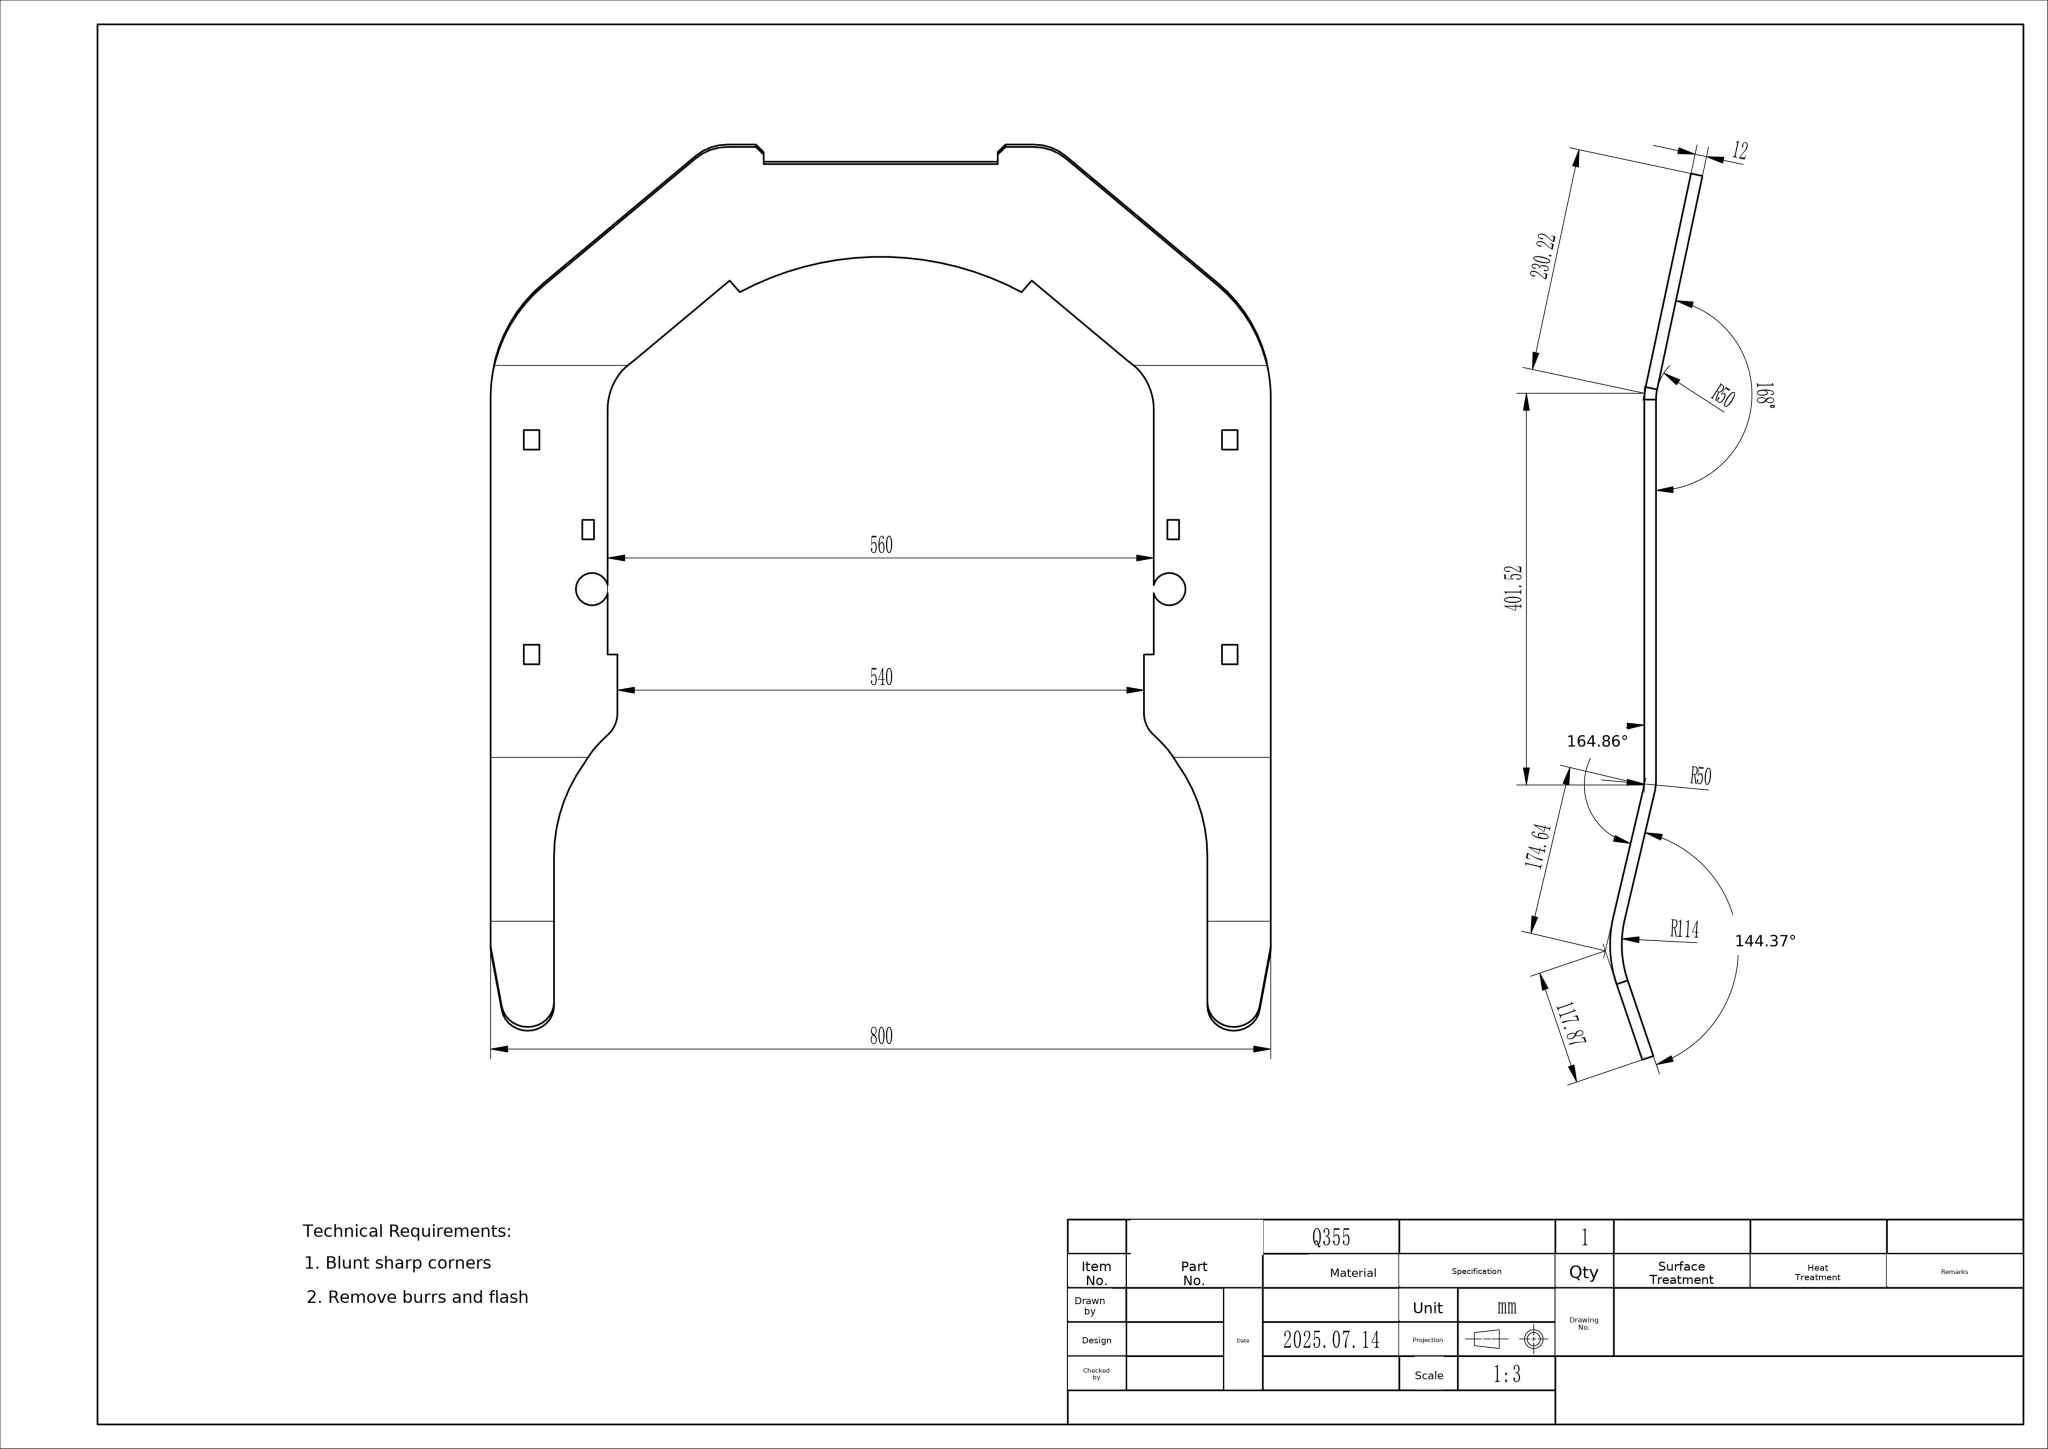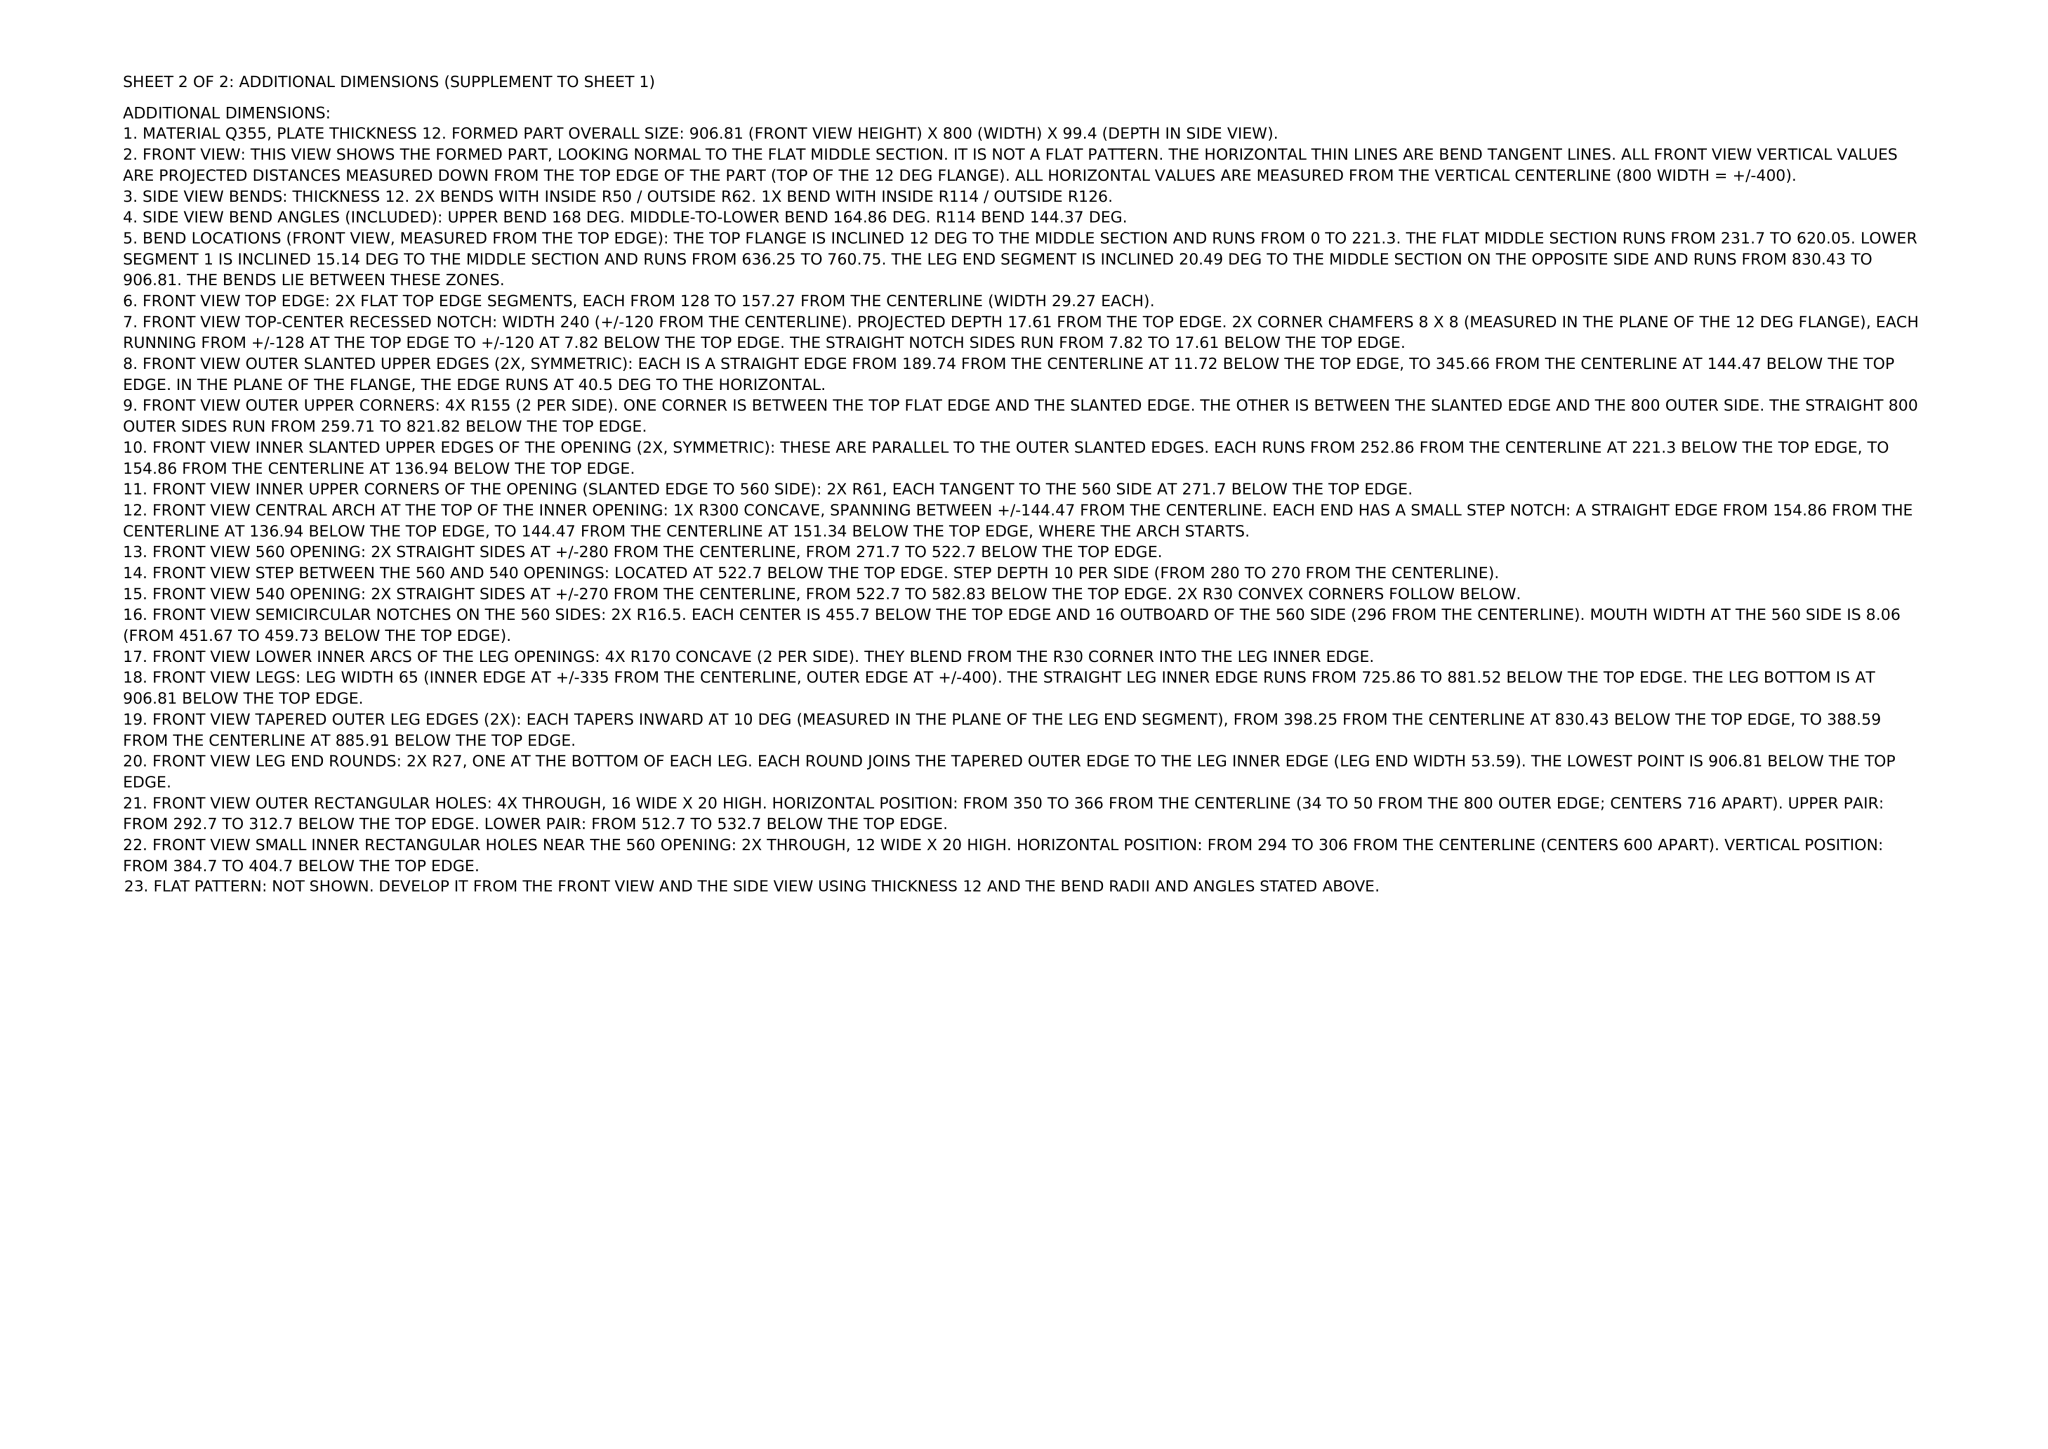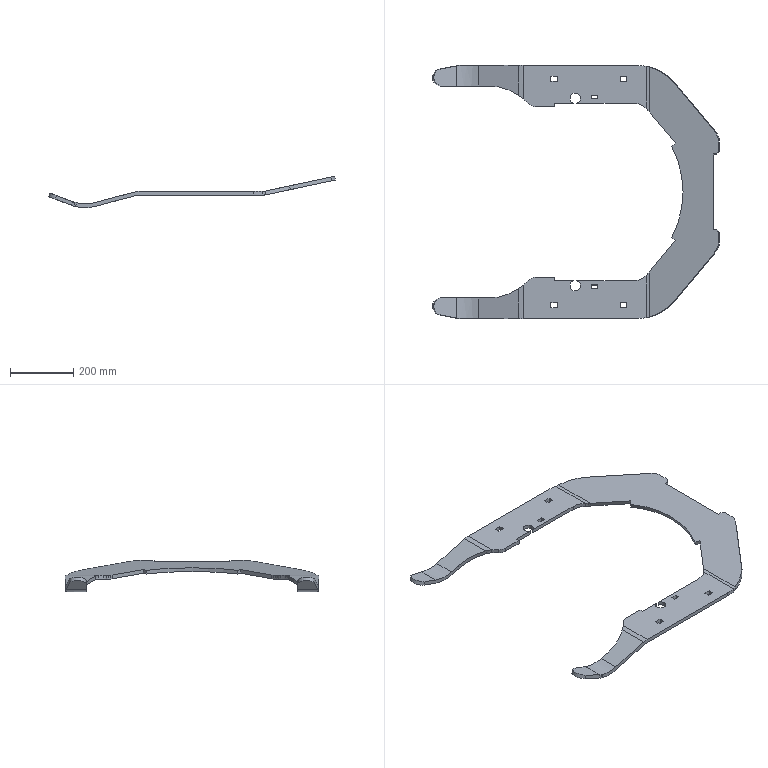Part | NX | mm | 1 solid | 108 faces | box 906.81 x 800 x 99.4 mm | volume 2718600 mm3 | plane 65 | cylinder 31 | spline 12 | commonest cylinder face diameters 100 x6 310 x4 340 x4 124 x4 33 x2 122 x2 60 x2 54 x2